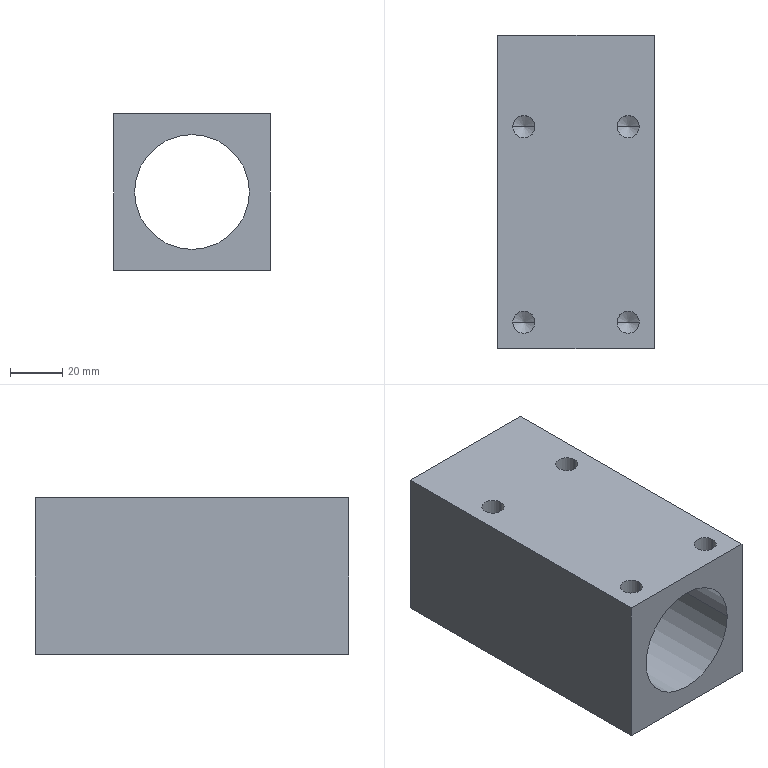Component | SolidWorks | -MovingBushing-3 | 1 solid | 40 faces | box 60 x 120 x 60 mm | volume 242794 mm3 | cylinder 18 | cone 16 | plane 6 | commonest cylinder face diameters 8.5 x16 44 x2
build123d program:
from build123d import *

# Parameters (mm, degrees)
SKETCH1_W                   = 60
SKETCH1_H                   = 60
SKETCH1_R                   = 22
BOSS_EXTRUDE1_DEPTH         = 60
M10_TAPPED_HOLE1_AT_2_COUNT = 2
M10_TAPPED_HOLE1_AT_2_PITCH = 40
M10_TAPPED_HOLE1_AT_3_COUNT = 2
M10_TAPPED_HOLE1_AT_3_PITCH = 75
M10_TAPPED_HOLE1_AT_4_COUNT = 2
M10_TAPPED_HOLE1_AT_4_PITCH = 85


with BuildPart() as part:
    # Sketch1 → Boss-Extrude1 (new, symmetric)
    with BuildSketch(Plane(origin=(0, 0, 0), x_dir=(0, 0, -1), z_dir=(1, 0, 0))):
        Rectangle(SKETCH1_W, SKETCH1_H)
        Circle(SKETCH1_R, mode=Mode.SUBTRACT)
    extrude(amount=BOSS_EXTRUDE1_DEPTH, both=True)

    # Sketch2 → M10 Tapped Hole1 (revolve, cut)
    with BuildSketch(Plane(origin=(-25, -30, 20), x_dir=(0, 0, -1), z_dir=(1, 0, 0))):
        Polygon((0, 0), (0, 16.554), (4.25, 14), (4.25, 0), align=None)
    m10_tapped_hole1 = revolve(axis=Axis((-25, -36.35, 20), (0, 1, 0)), mode=Mode.SUBTRACT)

    # M10 Tapped Hole1 at 2: M10 Tapped Hole1 ×2
    with Locations(*[(0, 0, -i * M10_TAPPED_HOLE1_AT_2_PITCH) for i in range(1, M10_TAPPED_HOLE1_AT_2_COUNT)]):
        add(m10_tapped_hole1, mode=Mode.SUBTRACT)

    # M10 Tapped Hole1 at 3: M10 Tapped Hole1 ×2
    with Locations(*[(i * M10_TAPPED_HOLE1_AT_3_PITCH, 0, 0) for i in range(1, M10_TAPPED_HOLE1_AT_3_COUNT)]):
        add(m10_tapped_hole1, mode=Mode.SUBTRACT)

    # M10 Tapped Hole1 at 4: M10 Tapped Hole1 ×2
    with Locations(*[Vector(0.8824, 0, -0.4706) * (i * M10_TAPPED_HOLE1_AT_4_PITCH) for i in range(1, M10_TAPPED_HOLE1_AT_4_COUNT)]):
        add(m10_tapped_hole1, mode=Mode.SUBTRACT)

    # Mirror1: M10 Tapped Hole1 across plane
    add(m10_tapped_hole1.mirror(Plane.ZX), mode=Mode.SUBTRACT)

    # Mirror1 copy 1 sketch → Mirror1 copy 1 (revolve, cut)
    with BuildSketch(Plane(origin=(-25, 30, -20), x_dir=(0, 0, -1), z_dir=(1, 0, 0))):
        Polygon((0, 0), (0, -16.554), (4.25, -14), (4.25, 0), align=None)
    revolve(axis=Axis((-25, 36.35, -20), (0, 1, 0)), mode=Mode.SUBTRACT)

    # Mirror1 copy 2 sketch → Mirror1 copy 2 (revolve, cut)
    with BuildSketch(Plane(origin=(50, 30, 20), x_dir=(0, 0, -1), z_dir=(1, 0, 0))):
        Polygon((0, 0), (0, -16.554), (4.25, -14), (4.25, 0), align=None)
    revolve(axis=Axis((50, 36.35, 20), (0, 1, 0)), mode=Mode.SUBTRACT)

    # Mirror1 copy 3 sketch → Mirror1 copy 3 (revolve, cut)
    with BuildSketch(Plane(origin=(50, 30, -20), x_dir=(0, 0, -1), z_dir=(1, 0, 0))):
        Polygon((0, 0), (0, -16.554), (4.25, -14), (4.25, 0), align=None)
    revolve(axis=Axis((50, 36.35, -20), (0, 1, 0)), mode=Mode.SUBTRACT)


solid = part.part

# Placed as in the assembly
solid = solid.moved(Location((-55, 1249.5, -40), (90, -90, 0)))
STEP:
#1=COLOUR_RGB('',0.7922,0.8196,0.9333);
#2=FILL_AREA_STYLE_COLOUR('',#1);
#3=FILL_AREA_STYLE('',(#2));
#4=SURFACE_STYLE_FILL_AREA(#3);
#5=SURFACE_SIDE_STYLE('',(#4));
#6=SURFACE_STYLE_USAGE(.BOTH.,#5);
#7=PRESENTATION_STYLE_ASSIGNMENT((#6));
#8=CARTESIAN_POINT('',(-1.545,50.177,-2.205));
#9=VERTEX_POINT('',#8);
#10=CARTESIAN_POINT('',(-1.211,50.177,-2.205));
#11=VERTEX_POINT('',#10);
#12=CARTESIAN_POINT('',(-1.378,50.177,-2.205));
#13=DIRECTION('',(-0.,-0.,-1.));
#14=DIRECTION('',(1.,0.,0.));
#15=AXIS2_PLACEMENT_3D('',#12,#13,#14);
#16=CIRCLE('',#15,0.1673);
#17=EDGE_CURVE('',#9,#11,#16,.T.);
#18=ORIENTED_EDGE('',*,*,#17,.F.);
#19=CARTESIAN_POINT('',(-1.545,50.177,-2.756));
#20=VERTEX_POINT('',#19);
#21=CARTESIAN_POINT('',(-1.545,50.177,-2.756));
#22=DIRECTION('',(-0.,-0.,-1.));
#23=VECTOR('',#22,39.37);
#24=LINE('',#21,#23);
#25=EDGE_CURVE('',#9,#20,#24,.T.);
#26=ORIENTED_EDGE('',*,*,#25,.T.);
#27=CARTESIAN_POINT('',(-1.211,50.177,-2.756));
#28=VERTEX_POINT('',#27);
#29=CARTESIAN_POINT('',(-1.378,50.177,-2.756));
#30=DIRECTION('',(-0.,-0.,-1.));
#31=DIRECTION('',(1.,0.,0.));
#32=AXIS2_PLACEMENT_3D('',#29,#30,#31);
#33=CIRCLE('',#32,0.1673);
#34=EDGE_CURVE('',#20,#28,#33,.T.);
#35=ORIENTED_EDGE('',*,*,#34,.T.);
#36=CARTESIAN_POINT('',(-1.211,50.177,-2.756));
#37=DIRECTION('',(-0.,-0.,-1.));
#38=VECTOR('',#37,39.37);
#39=LINE('',#36,#38);
#40=EDGE_CURVE('',#11,#28,#39,.T.);
#41=ORIENTED_EDGE('',*,*,#40,.F.);
#42=EDGE_LOOP('',(#18,#26,#35,#41));
#43=FACE_OUTER_BOUND('',#42,.T.);
#44=CARTESIAN_POINT('',(-1.378,50.177,-2.756));
#45=DIRECTION('',(-0.,-0.,-1.));
#46=DIRECTION('',(1.,0.,0.));
#47=AXIS2_PLACEMENT_3D('',#44,#45,#46);
#48=CYLINDRICAL_SURFACE('',#47,0.1673);
#49=ADVANCED_FACE('',(#43),#48,.F.);
#50=CARTESIAN_POINT('',(-1.378,50.177,-2.104));
#51=VERTEX_POINT('',#50);
#52=CARTESIAN_POINT('',(-1.211,50.177,-2.205));
#53=DIRECTION('',(0.8572,0.,-0.515));
#54=VECTOR('',#53,39.37);
#55=LINE('',#52,#54);
#56=EDGE_CURVE('',#51,#11,#55,.T.);
#57=ORIENTED_EDGE('',*,*,#56,.F.);
#58=CARTESIAN_POINT('',(-1.545,50.177,-2.205));
#59=DIRECTION('',(-0.8572,-0.,-0.515));
#60=VECTOR('',#59,39.37);
#61=LINE('',#58,#60);
#62=EDGE_CURVE('',#51,#9,#61,.T.);
#63=ORIENTED_EDGE('',*,*,#62,.T.);
#64=ORIENTED_EDGE('',*,*,#17,.T.);
#65=EDGE_LOOP('',(#57,#63,#64));
#66=FACE_OUTER_BOUND('',#65,.T.);
#67=CARTESIAN_POINT('',(-1.378,50.177,-2.205));
#68=DIRECTION('',(-0.,-0.,-1.));
#69=DIRECTION('',(1.,0.,0.));
#70=AXIS2_PLACEMENT_3D('',#67,#68,#69);
#71=CONICAL_SURFACE('',#70,0.1673,1.03);
#72=ADVANCED_FACE('',(#66),#71,.F.);
#73=CARTESIAN_POINT('',(-3.12,50.177,-2.205));
#74=VERTEX_POINT('',#73);
#75=CARTESIAN_POINT('',(-2.785,50.177,-2.205));
#76=VERTEX_POINT('',#75);
#77=CARTESIAN_POINT('',(-2.953,50.177,-2.205));
#78=DIRECTION('',(-0.,-0.,-1.));
#79=DIRECTION('',(1.,0.,0.));
#80=AXIS2_PLACEMENT_3D('',#77,#78,#79);
#81=CIRCLE('',#80,0.1673);
#82=EDGE_CURVE('',#74,#76,#81,.T.);
#83=ORIENTED_EDGE('',*,*,#82,.F.);
#84=CARTESIAN_POINT('',(-3.12,50.177,-2.756));
#85=VERTEX_POINT('',#84);
#86=CARTESIAN_POINT('',(-3.12,50.177,-2.756));
#87=DIRECTION('',(-0.,-0.,-1.));
#88=VECTOR('',#87,39.37);
#89=LINE('',#86,#88);
#90=EDGE_CURVE('',#74,#85,#89,.T.);
#91=ORIENTED_EDGE('',*,*,#90,.T.);
#92=CARTESIAN_POINT('',(-2.785,50.177,-2.756));
#93=VERTEX_POINT('',#92);
#94=CARTESIAN_POINT('',(-2.953,50.177,-2.756));
#95=DIRECTION('',(-0.,-0.,-1.));
#96=DIRECTION('',(1.,0.,0.));
#97=AXIS2_PLACEMENT_3D('',#94,#95,#96);
#98=CIRCLE('',#97,0.1673);
#99=EDGE_CURVE('',#85,#93,#98,.T.);
#100=ORIENTED_EDGE('',*,*,#99,.T.);
#101=CARTESIAN_POINT('',(-2.785,50.177,-2.756));
#102=DIRECTION('',(-0.,-0.,-1.));
#103=VECTOR('',#102,39.37);
#104=LINE('',#101,#103);
#105=EDGE_CURVE('',#76,#93,#104,.T.);
#106=ORIENTED_EDGE('',*,*,#105,.F.);
#107=EDGE_LOOP('',(#83,#91,#100,#106));
#108=FACE_OUTER_BOUND('',#107,.T.);
#109=CARTESIAN_POINT('',(-2.953,50.177,-2.756));
#110=DIRECTION('',(-0.,-0.,-1.));
#111=DIRECTION('',(1.,0.,0.));
#112=AXIS2_PLACEMENT_3D('',#109,#110,#111);
#113=CYLINDRICAL_SURFACE('',#112,0.1673);
#114=ADVANCED_FACE('',(#108),#113,.F.);
#115=CARTESIAN_POINT('',(-2.953,50.177,-2.104));
#116=VERTEX_POINT('',#115);
#117=CARTESIAN_POINT('',(-2.785,50.177,-2.205));
#118=DIRECTION('',(0.8572,0.,-0.515));
#119=VECTOR('',#118,39.37);
#120=LINE('',#117,#119);
#121=EDGE_CURVE('',#116,#76,#120,.T.);
#122=ORIENTED_EDGE('',*,*,#121,.F.);
#123=CARTESIAN_POINT('',(-3.12,50.177,-2.205));
#124=DIRECTION('',(-0.8572,-0.,-0.515));
#125=VECTOR('',#124,39.37);
#126=LINE('',#123,#125);
#127=EDGE_CURVE('',#116,#74,#126,.T.);
#128=ORIENTED_EDGE('',*,*,#127,.T.);
#129=ORIENTED_EDGE('',*,*,#82,.T.);
#130=EDGE_LOOP('',(#122,#128,#129));
#131=FACE_OUTER_BOUND('',#130,.T.);
#132=CARTESIAN_POINT('',(-2.953,50.177,-2.205));
#133=DIRECTION('',(-0.,-0.,-1.));
#134=DIRECTION('',(1.,0.,0.));
#135=AXIS2_PLACEMENT_3D('',#132,#133,#134);
#136=CONICAL_SURFACE('',#135,0.1673,1.03);
#137=ADVANCED_FACE('',(#131),#136,.F.);
#138=CARTESIAN_POINT('',(-1.545,47.224,-2.205));
#139=VERTEX_POINT('',#138);
#140=CARTESIAN_POINT('',(-1.211,47.224,-2.205));
#141=VERTEX_POINT('',#140);
#142=CARTESIAN_POINT('',(-1.378,47.224,-2.205));
#143=DIRECTION('',(-0.,-0.,-1.));
#144=DIRECTION('',(1.,0.,0.));
#145=AXIS2_PLACEMENT_3D('',#142,#143,#144);
#146=CIRCLE('',#145,0.1673);
#147=EDGE_CURVE('',#139,#141,#146,.T.);
#148=ORIENTED_EDGE('',*,*,#147,.F.);
#149=CARTESIAN_POINT('',(-1.545,47.224,-2.756));
#150=VERTEX_POINT('',#149);
#151=CARTESIAN_POINT('',(-1.545,47.224,-2.756));
#152=DIRECTION('',(-0.,-0.,-1.));
#153=VECTOR('',#152,39.37);
#154=LINE('',#151,#153);
#155=EDGE_CURVE('',#139,#150,#154,.T.);
#156=ORIENTED_EDGE('',*,*,#155,.T.);
#157=CARTESIAN_POINT('',(-1.211,47.224,-2.756));
#158=VERTEX_POINT('',#157);
#159=CARTESIAN_POINT('',(-1.378,47.224,-2.756));
#160=DIRECTION('',(-0.,-0.,-1.));
#161=DIRECTION('',(1.,0.,0.));
#162=AXIS2_PLACEMENT_3D('',#159,#160,#161);
#163=CIRCLE('',#162,0.1673);
#164=EDGE_CURVE('',#150,#158,#163,.T.);
#165=ORIENTED_EDGE('',*,*,#164,.T.);
#166=CARTESIAN_POINT('',(-1.211,47.224,-2.756));
#167=DIRECTION('',(-0.,-0.,-1.));
#168=VECTOR('',#167,39.37);
#169=LINE('',#166,#168);
#170=EDGE_CURVE('',#141,#158,#169,.T.);
#171=ORIENTED_EDGE('',*,*,#170,.F.);
#172=EDGE_LOOP('',(#148,#156,#165,#171));
#173=FACE_OUTER_BOUND('',#172,.T.);
#174=CARTESIAN_POINT('',(-1.378,47.224,-2.756));
#175=DIRECTION('',(-0.,-0.,-1.));
#176=DIRECTION('',(1.,0.,0.));
#177=AXIS2_PLACEMENT_3D('',#174,#175,#176);
#178=CYLINDRICAL_SURFACE('',#177,0.1673);
#179=ADVANCED_FACE('',(#173),#178,.F.);
#180=CARTESIAN_POINT('',(-1.378,47.224,-2.104));
#181=VERTEX_POINT('',#180);
#182=CARTESIAN_POINT('',(-1.211,47.224,-2.205));
#183=DIRECTION('',(0.8572,0.,-0.515));
#184=VECTOR('',#183,39.37);
#185=LINE('',#182,#184);
#186=EDGE_CURVE('',#181,#141,#185,.T.);
#187=ORIENTED_EDGE('',*,*,#186,.F.);
#188=CARTESIAN_POINT('',(-1.545,47.224,-2.205));
#189=DIRECTION('',(-0.8572,-0.,-0.515));
#190=VECTOR('',#189,39.37);
#191=LINE('',#188,#190);
#192=EDGE_CURVE('',#181,#139,#191,.T.);
#193=ORIENTED_EDGE('',*,*,#192,.T.);
#194=ORIENTED_EDGE('',*,*,#147,.T.);
#195=EDGE_LOOP('',(#187,#193,#194));
#196=FACE_OUTER_BOUND('',#195,.T.);
#197=CARTESIAN_POINT('',(-1.378,47.224,-2.205));
#198=DIRECTION('',(-0.,-0.,-1.));
#199=DIRECTION('',(1.,0.,0.));
#200=AXIS2_PLACEMENT_3D('',#197,#198,#199);
#201=CONICAL_SURFACE('',#200,0.1673,1.03);
#202=ADVANCED_FACE('',(#196),#201,.F.);
#203=CARTESIAN_POINT('',(-3.12,47.224,-2.205));
#204=VERTEX_POINT('',#203);
#205=CARTESIAN_POINT('',(-2.785,47.224,-2.205));
#206=VERTEX_POINT('',#205);
#207=CARTESIAN_POINT('',(-2.953,47.224,-2.205));
#208=DIRECTION('',(-0.,-0.,-1.));
#209=DIRECTION('',(1.,0.,0.));
#210=AXIS2_PLACEMENT_3D('',#207,#208,#209);
#211=CIRCLE('',#210,0.1673);
#212=EDGE_CURVE('',#204,#206,#211,.T.);
#213=ORIENTED_EDGE('',*,*,#212,.F.);
#214=CARTESIAN_POINT('',(-3.12,47.224,-2.756));
#215=VERTEX_POINT('',#214);
#216=CARTESIAN_POINT('',(-3.12,47.224,-2.756));
#217=DIRECTION('',(-0.,-0.,-1.));
#218=VECTOR('',#217,39.37);
#219=LINE('',#216,#218);
#220=EDGE_CURVE('',#204,#215,#219,.T.);
#221=ORIENTED_EDGE('',*,*,#220,.T.);
#222=CARTESIAN_POINT('',(-2.785,47.224,-2.756));
#223=VERTEX_POINT('',#222);
#224=CARTESIAN_POINT('',(-2.953,47.224,-2.756));
#225=DIRECTION('',(-0.,-0.,-1.));
#226=DIRECTION('',(1.,0.,0.));
#227=AXIS2_PLACEMENT_3D('',#224,#225,#226);
#228=CIRCLE('',#227,0.1673);
#229=EDGE_CURVE('',#215,#223,#228,.T.);
#230=ORIENTED_EDGE('',*,*,#229,.T.);
#231=CARTESIAN_POINT('',(-2.785,47.224,-2.756));
#232=DIRECTION('',(-0.,-0.,-1.));
#233=VECTOR('',#232,39.37);
#234=LINE('',#231,#233);
#235=EDGE_CURVE('',#206,#223,#234,.T.);
#236=ORIENTED_EDGE('',*,*,#235,.F.);
#237=EDGE_LOOP('',(#213,#221,#230,#236));
#238=FACE_OUTER_BOUND('',#237,.T.);
#239=CARTESIAN_POINT('',(-2.953,47.224,-2.756));
#240=DIRECTION('',(-0.,-0.,-1.));
#241=DIRECTION('',(1.,0.,0.));
#242=AXIS2_PLACEMENT_3D('',#239,#240,#241);
#243=CYLINDRICAL_SURFACE('',#242,0.1673);
#244=ADVANCED_FACE('',(#238),#243,.F.);
#245=CARTESIAN_POINT('',(-2.953,47.224,-2.104));
#246=VERTEX_POINT('',#245);
#247=CARTESIAN_POINT('',(-2.785,47.224,-2.205));
#248=DIRECTION('',(0.8572,0.,-0.515));
#249=VECTOR('',#248,39.37);
#250=LINE('',#247,#249);
#251=EDGE_CURVE('',#246,#206,#250,.T.);
#252=ORIENTED_EDGE('',*,*,#251,.F.);
#253=CARTESIAN_POINT('',(-3.12,47.224,-2.205));
#254=DIRECTION('',(-0.8572,-0.,-0.515));
#255=VECTOR('',#254,39.37);
#256=LINE('',#253,#255);
#257=EDGE_CURVE('',#246,#204,#256,.T.);
#258=ORIENTED_EDGE('',*,*,#257,.T.);
#259=ORIENTED_EDGE('',*,*,#212,.T.);
#260=EDGE_LOOP('',(#252,#258,#259));
#261=FACE_OUTER_BOUND('',#260,.T.);
#262=CARTESIAN_POINT('',(-2.953,47.224,-2.205));
#263=DIRECTION('',(-0.,-0.,-1.));
#264=DIRECTION('',(1.,0.,0.));
#265=AXIS2_PLACEMENT_3D('',#262,#263,#264);
#266=CONICAL_SURFACE('',#265,0.1673,1.03);
#267=ADVANCED_FACE('',(#261),#266,.F.);
#268=CARTESIAN_POINT('',(-1.211,50.177,-0.9449));
#269=VERTEX_POINT('',#268);
#270=CARTESIAN_POINT('',(-1.545,50.177,-0.9449));
#271=VERTEX_POINT('',#270);
#272=CARTESIAN_POINT('',(-1.378,50.177,-0.9449));
#273=DIRECTION('',(0.,0.,1.));
#274=DIRECTION('',(-1.,0.,0.));
#275=AXIS2_PLACEMENT_3D('',#272,#273,#274);
#276=CIRCLE('',#275,0.1673);
#277=EDGE_CURVE('',#269,#271,#276,.T.);
#278=ORIENTED_EDGE('',*,*,#277,.F.);
#279=CARTESIAN_POINT('',(-1.211,50.177,-0.3937));
#280=VERTEX_POINT('',#279);
#281=CARTESIAN_POINT('',(-1.211,50.177,-0.3937));
#282=DIRECTION('',(0.,0.,1.));
#283=VECTOR('',#282,39.37);
#284=LINE('',#281,#283);
#285=EDGE_CURVE('',#269,#280,#284,.T.);
#286=ORIENTED_EDGE('',*,*,#285,.T.);
#287=CARTESIAN_POINT('',(-1.545,50.177,-0.3937));
#288=VERTEX_POINT('',#287);
#289=CARTESIAN_POINT('',(-1.378,50.177,-0.3937));
#290=DIRECTION('',(0.,0.,1.));
#291=DIRECTION('',(-1.,0.,0.));
#292=AXIS2_PLACEMENT_3D('',#289,#290,#291);
#293=CIRCLE('',#292,0.1673);
#294=EDGE_CURVE('',#280,#288,#293,.T.);
#295=ORIENTED_EDGE('',*,*,#294,.T.);
#296=CARTESIAN_POINT('',(-1.545,50.177,-0.3937));
#297=DIRECTION('',(0.,0.,1.));
#298=VECTOR('',#297,39.37);
#299=LINE('',#296,#298);
#300=EDGE_CURVE('',#271,#288,#299,.T.);
#301=ORIENTED_EDGE('',*,*,#300,.F.);
#302=EDGE_LOOP('',(#278,#286,#295,#301));
#303=FACE_OUTER_BOUND('',#302,.T.);
#304=CARTESIAN_POINT('',(-1.378,50.177,-0.3937));
#305=DIRECTION('',(0.,0.,1.));
#306=DIRECTION('',(-1.,0.,0.));
#307=AXIS2_PLACEMENT_3D('',#304,#305,#306);
#308=CYLINDRICAL_SURFACE('',#307,0.1673);
#309=ADVANCED_FACE('',(#303),#308,.F.);
#310=CARTESIAN_POINT('',(-1.378,50.177,-1.045));
#311=VERTEX_POINT('',#310);
#312=CARTESIAN_POINT('',(-1.545,50.177,-0.9449));
#313=DIRECTION('',(-0.8572,-0.,0.515));
#314=VECTOR('',#313,39.37);
#315=LINE('',#312,#314);
#316=EDGE_CURVE('',#311,#271,#315,.T.);
#317=ORIENTED_EDGE('',*,*,#316,.F.);
#318=CARTESIAN_POINT('',(-1.211,50.177,-0.9449));
#319=DIRECTION('',(0.8572,0.,0.515));
#320=VECTOR('',#319,39.37);
#321=LINE('',#318,#320);
#322=EDGE_CURVE('',#311,#269,#321,.T.);
#323=ORIENTED_EDGE('',*,*,#322,.T.);
#324=ORIENTED_EDGE('',*,*,#277,.T.);
#325=EDGE_LOOP('',(#317,#323,#324));
#326=FACE_OUTER_BOUND('',#325,.T.);
#327=CARTESIAN_POINT('',(-1.378,50.177,-0.9449));
#328=DIRECTION('',(0.,0.,1.));
#329=DIRECTION('',(-1.,0.,0.));
#330=AXIS2_PLACEMENT_3D('',#327,#328,#329);
#331=CONICAL_SURFACE('',#330,0.1673,1.03);
#332=ADVANCED_FACE('',(#326),#331,.F.);
#333=CARTESIAN_POINT('',(-2.785,50.177,-0.9449));
#334=VERTEX_POINT('',#333);
#335=CARTESIAN_POINT('',(-3.12,50.177,-0.9449));
#336=VERTEX_POINT('',#335);
#337=CARTESIAN_POINT('',(-2.953,50.177,-0.9449));
#338=DIRECTION('',(0.,0.,1.));
#339=DIRECTION('',(-1.,0.,0.));
#340=AXIS2_PLACEMENT_3D('',#337,#338,#339);
#341=CIRCLE('',#340,0.1673);
#342=EDGE_CURVE('',#334,#336,#341,.T.);
#343=ORIENTED_EDGE('',*,*,#342,.F.);
#344=CARTESIAN_POINT('',(-2.785,50.177,-0.3937));
#345=VERTEX_POINT('',#344);
#346=CARTESIAN_POINT('',(-2.785,50.177,-0.3937));
#347=DIRECTION('',(0.,0.,1.));
#348=VECTOR('',#347,39.37);
#349=LINE('',#346,#348);
#350=EDGE_CURVE('',#334,#345,#349,.T.);
#351=ORIENTED_EDGE('',*,*,#350,.T.);
#352=CARTESIAN_POINT('',(-3.12,50.177,-0.3937));
#353=VERTEX_POINT('',#352);
#354=CARTESIAN_POINT('',(-2.953,50.177,-0.3937));
#355=DIRECTION('',(0.,0.,1.));
#356=DIRECTION('',(-1.,0.,0.));
#357=AXIS2_PLACEMENT_3D('',#354,#355,#356);
#358=CIRCLE('',#357,0.1673);
#359=EDGE_CURVE('',#345,#353,#358,.T.);
#360=ORIENTED_EDGE('',*,*,#359,.T.);
#361=CARTESIAN_POINT('',(-3.12,50.177,-0.3937));
#362=DIRECTION('',(0.,0.,1.));
#363=VECTOR('',#362,39.37);
#364=LINE('',#361,#363);
#365=EDGE_CURVE('',#336,#353,#364,.T.);
#366=ORIENTED_EDGE('',*,*,#365,.F.);
#367=EDGE_LOOP('',(#343,#351,#360,#366));
#368=FACE_OUTER_BOUND('',#367,.T.);
#369=CARTESIAN_POINT('',(-2.953,50.177,-0.3937));
#370=DIRECTION('',(0.,0.,1.));
#371=DIRECTION('',(-1.,0.,0.));
#372=AXIS2_PLACEMENT_3D('',#369,#370,#371);
#373=CYLINDRICAL_SURFACE('',#372,0.1673);
#374=ADVANCED_FACE('',(#368),#373,.F.);
#375=CARTESIAN_POINT('',(-2.953,50.177,-1.045));
#376=VERTEX_POINT('',#375);
#377=CARTESIAN_POINT('',(-3.12,50.177,-0.9449));
#378=DIRECTION('',(-0.8572,-0.,0.515));
#379=VECTOR('',#378,39.37);
#380=LINE('',#377,#379);
#381=EDGE_CURVE('',#376,#336,#380,.T.);
#382=ORIENTED_EDGE('',*,*,#381,.F.);
#383=CARTESIAN_POINT('',(-2.785,50.177,-0.9449));
#384=DIRECTION('',(0.8572,0.,0.515));
#385=VECTOR('',#384,39.37);
#386=LINE('',#383,#385);
#387=EDGE_CURVE('',#376,#334,#386,.T.);
#388=ORIENTED_EDGE('',*,*,#387,.T.);
#389=ORIENTED_EDGE('',*,*,#342,.T.);
#390=EDGE_LOOP('',(#382,#388,#389));
#391=FACE_OUTER_BOUND('',#390,.T.);
#392=CARTESIAN_POINT('',(-2.953,50.177,-0.9449));
#393=DIRECTION('',(0.,0.,1.));
#394=DIRECTION('',(-1.,0.,0.));
#395=AXIS2_PLACEMENT_3D('',#392,#393,#394);
#396=CONICAL_SURFACE('',#395,0.1673,1.03);
#397=ADVANCED_FACE('',(#391),#396,.F.);
#398=CARTESIAN_POINT('',(-1.211,47.224,-0.9449));
#399=VERTEX_POINT('',#398);
#400=CARTESIAN_POINT('',(-1.545,47.224,-0.9449));
#401=VERTEX_POINT('',#400);
#402=CARTESIAN_POINT('',(-1.378,47.224,-0.9449));
#403=DIRECTION('',(0.,0.,1.));
#404=DIRECTION('',(-1.,0.,0.));
#405=AXIS2_PLACEMENT_3D('',#402,#403,#404);
#406=CIRCLE('',#405,0.1673);
#407=EDGE_CURVE('',#399,#401,#406,.T.);
#408=ORIENTED_EDGE('',*,*,#407,.F.);
#409=CARTESIAN_POINT('',(-1.211,47.224,-0.3937));
#410=VERTEX_POINT('',#409);
#411=CARTESIAN_POINT('',(-1.211,47.224,-0.3937));
#412=DIRECTION('',(0.,0.,1.));
#413=VECTOR('',#412,39.37);
#414=LINE('',#411,#413);
#415=EDGE_CURVE('',#399,#410,#414,.T.);
#416=ORIENTED_EDGE('',*,*,#415,.T.);
#417=CARTESIAN_POINT('',(-1.545,47.224,-0.3937));
#418=VERTEX_POINT('',#417);
#419=CARTESIAN_POINT('',(-1.378,47.224,-0.3937));
#420=DIRECTION('',(0.,0.,1.));
#421=DIRECTION('',(-1.,0.,0.));
#422=AXIS2_PLACEMENT_3D('',#419,#420,#421);
#423=CIRCLE('',#422,0.1673);
#424=EDGE_CURVE('',#410,#418,#423,.T.);
#425=ORIENTED_EDGE('',*,*,#424,.T.);
#426=CARTESIAN_POINT('',(-1.545,47.224,-0.3937));
#427=DIRECTION('',(0.,0.,1.));
#428=VECTOR('',#427,39.37);
#429=LINE('',#426,#428);
#430=EDGE_CURVE('',#401,#418,#429,.T.);
#431=ORIENTED_EDGE('',*,*,#430,.F.);
#432=EDGE_LOOP('',(#408,#416,#425,#431));
#433=FACE_OUTER_BOUND('',#432,.T.);
#434=CARTESIAN_POINT('',(-1.378,47.224,-0.3937));
#435=DIRECTION('',(0.,0.,1.));
#436=DIRECTION('',(-1.,0.,0.));
#437=AXIS2_PLACEMENT_3D('',#434,#435,#436);
#438=CYLINDRICAL_SURFACE('',#437,0.1673);
#439=ADVANCED_FACE('',(#433),#438,.F.);
#440=CARTESIAN_POINT('',(-1.378,47.224,-1.045));
#441=VERTEX_POINT('',#440);
#442=CARTESIAN_POINT('',(-1.545,47.224,-0.9449));
#443=DIRECTION('',(-0.8572,-0.,0.515));
#444=VECTOR('',#443,39.37);
#445=LINE('',#442,#444);
#446=EDGE_CURVE('',#441,#401,#445,.T.);
#447=ORIENTED_EDGE('',*,*,#446,.F.);
#448=CARTESIAN_POINT('',(-1.211,47.224,-0.9449));
#449=DIRECTION('',(0.8572,0.,0.515));
#450=VECTOR('',#449,39.37);
#451=LINE('',#448,#450);
#452=EDGE_CURVE('',#441,#399,#451,.T.);
#453=ORIENTED_EDGE('',*,*,#452,.T.);
#454=ORIENTED_EDGE('',*,*,#407,.T.);
#455=EDGE_LOOP('',(#447,#453,#454));
#456=FACE_OUTER_BOUND('',#455,.T.);
#457=CARTESIAN_POINT('',(-1.378,47.224,-0.9449));
#458=DIRECTION('',(0.,0.,1.));
#459=DIRECTION('',(-1.,0.,0.));
#460=AXIS2_PLACEMENT_3D('',#457,#458,#459);
#461=CONICAL_SURFACE('',#460,0.1673,1.03);
#462=ADVANCED_FACE('',(#456),#461,.F.);
#463=CARTESIAN_POINT('',(-2.785,47.224,-0.9449));
#464=VERTEX_POINT('',#463);
#465=CARTESIAN_POINT('',(-3.12,47.224,-0.9449));
#466=VERTEX_POINT('',#465);
#467=CARTESIAN_POINT('',(-2.953,47.224,-0.9449));
#468=DIRECTION('',(0.,0.,1.));
#469=DIRECTION('',(-1.,0.,0.));
#470=AXIS2_PLACEMENT_3D('',#467,#468,#469);
#471=CIRCLE('',#470,0.1673);
#472=EDGE_CURVE('',#464,#466,#471,.T.);
#473=ORIENTED_EDGE('',*,*,#472,.F.);
#474=CARTESIAN_POINT('',(-2.785,47.224,-0.3937));
#475=VERTEX_POINT('',#474);
#476=CARTESIAN_POINT('',(-2.785,47.224,-0.3937));
#477=DIRECTION('',(0.,0.,1.));
#478=VECTOR('',#477,39.37);
#479=LINE('',#476,#478);
#480=EDGE_CURVE('',#464,#475,#479,.T.);
#481=ORIENTED_EDGE('',*,*,#480,.T.);
#482=CARTESIAN_POINT('',(-3.12,47.224,-0.3937));
#483=VERTEX_POINT('',#482);
#484=CARTESIAN_POINT('',(-2.953,47.224,-0.3937));
#485=DIRECTION('',(0.,0.,1.));
#486=DIRECTION('',(-1.,0.,0.));
#487=AXIS2_PLACEMENT_3D('',#484,#485,#486);
#488=CIRCLE('',#487,0.1673);
#489=EDGE_CURVE('',#475,#483,#488,.T.);
#490=ORIENTED_EDGE('',*,*,#489,.T.);
#491=CARTESIAN_POINT('',(-3.12,47.224,-0.3937));
#492=DIRECTION('',(0.,0.,1.));
#493=VECTOR('',#492,39.37);
#494=LINE('',#491,#493);
#495=EDGE_CURVE('',#466,#483,#494,.T.);
#496=ORIENTED_EDGE('',*,*,#495,.F.);
#497=EDGE_LOOP('',(#473,#481,#490,#496));
#498=FACE_OUTER_BOUND('',#497,.T.);
#499=CARTESIAN_POINT('',(-2.953,47.224,-0.3937));
#500=DIRECTION('',(0.,0.,1.));
#501=DIRECTION('',(-1.,0.,0.));
#502=AXIS2_PLACEMENT_3D('',#499,#500,#501);
#503=CYLINDRICAL_SURFACE('',#502,0.1673);
#504=ADVANCED_FACE('',(#498),#503,.F.);
#505=CARTESIAN_POINT('',(-2.953,47.224,-1.045));
#506=VERTEX_POINT('',#505);
#507=CARTESIAN_POINT('',(-3.12,47.224,-0.9449));
#508=DIRECTION('',(-0.8572,-0.,0.515));
#509=VECTOR('',#508,39.37);
#510=LINE('',#507,#509);
#511=EDGE_CURVE('',#506,#466,#510,.T.);
#512=ORIENTED_EDGE('',*,*,#511,.F.);
#513=CARTESIAN_POINT('',(-2.785,47.224,-0.9449));
#514=DIRECTION('',(0.8572,0.,0.515));
#515=VECTOR('',#514,39.37);
#516=LINE('',#513,#515);
#517=EDGE_CURVE('',#506,#464,#516,.T.);
#518=ORIENTED_EDGE('',*,*,#517,.T.);
#519=ORIENTED_EDGE('',*,*,#472,.T.);
#520=EDGE_LOOP('',(#512,#518,#519));
#521=FACE_OUTER_BOUND('',#520,.T.);
#522=CARTESIAN_POINT('',(-2.953,47.224,-0.9449));
#523=DIRECTION('',(0.,0.,1.));
#524=DIRECTION('',(-1.,0.,0.));
#525=AXIS2_PLACEMENT_3D('',#522,#523,#524);
#526=CONICAL_SURFACE('',#525,0.1673,1.03);
#527=ADVANCED_FACE('',(#521),#526,.F.);
#528=CARTESIAN_POINT('',(-1.299,46.831,-1.575));
#529=VERTEX_POINT('',#528);
#530=CARTESIAN_POINT('',(-3.031,46.831,-1.575));
#531=VERTEX_POINT('',#530);
#532=CARTESIAN_POINT('',(-2.165,46.831,-1.575));
#533=DIRECTION('',(0.,-1.,0.));
#534=DIRECTION('',(-1.,-0.,0.));
#535=AXIS2_PLACEMENT_3D('',#532,#533,#534);
#536=CIRCLE('',#535,0.8661);
#537=EDGE_CURVE('',#529,#531,#536,.T.);
#538=ORIENTED_EDGE('',*,*,#537,.T.);
#539=CARTESIAN_POINT('',(-3.031,51.555,-1.575));
#540=VERTEX_POINT('',#539);
#541=CARTESIAN_POINT('',(-3.031,46.831,-1.575));
#542=DIRECTION('',(-0.,1.,-0.));
#543=VECTOR('',#542,39.37);
#544=LINE('',#541,#543);
#545=EDGE_CURVE('',#531,#540,#544,.T.);
#546=ORIENTED_EDGE('',*,*,#545,.T.);
#547=CARTESIAN_POINT('',(-1.299,51.555,-1.575));
#548=VERTEX_POINT('',#547);
#549=CARTESIAN_POINT('',(-2.165,51.555,-1.575));
#550=DIRECTION('',(0.,-1.,0.));
#551=DIRECTION('',(-1.,-0.,0.));
#552=AXIS2_PLACEMENT_3D('',#549,#550,#551);
#553=CIRCLE('',#552,0.8661);
#554=EDGE_CURVE('',#548,#540,#553,.T.);
#555=ORIENTED_EDGE('',*,*,#554,.F.);
#556=CARTESIAN_POINT('',(-1.299,46.831,-1.575));
#557=DIRECTION('',(-0.,1.,-0.));
#558=VECTOR('',#557,39.37);
#559=LINE('',#556,#558);
#560=EDGE_CURVE('',#529,#548,#559,.T.);
#561=ORIENTED_EDGE('',*,*,#560,.F.);
#562=EDGE_LOOP('',(#538,#546,#555,#561));
#563=FACE_OUTER_BOUND('',#562,.T.);
#564=CARTESIAN_POINT('',(-2.165,46.831,-1.575));
#565=DIRECTION('',(-0.,1.,-0.));
#566=DIRECTION('',(1.,0.,-0.));
#567=AXIS2_PLACEMENT_3D('',#564,#565,#566);
#568=CYLINDRICAL_SURFACE('',#567,0.8661);
#569=ADVANCED_FACE('',(#563),#568,.F.);
#570=CARTESIAN_POINT('',(-3.346,46.831,-0.3937));
#571=VERTEX_POINT('',#570);
#572=CARTESIAN_POINT('',(-3.346,46.831,-2.756));
#573=VERTEX_POINT('',#572);
#574=CARTESIAN_POINT('',(-3.346,46.831,-2.756));
#575=DIRECTION('',(-0.,-0.,-1.));
#576=VECTOR('',#575,39.37);
#577=LINE('',#574,#576);
#578=EDGE_CURVE('',#571,#573,#577,.T.);
#579=ORIENTED_EDGE('',*,*,#578,.T.);
#580=CARTESIAN_POINT('',(-0.9843,46.831,-2.756));
#581=VERTEX_POINT('',#580);
#582=CARTESIAN_POINT('',(-0.9843,46.831,-2.756));
#583=DIRECTION('',(1.,0.,-0.));
#584=VECTOR('',#583,39.37);
#585=LINE('',#582,#584);
#586=EDGE_CURVE('',#573,#581,#585,.T.);
#587=ORIENTED_EDGE('',*,*,#586,.T.);
#588=CARTESIAN_POINT('',(-0.9843,46.831,-0.3937));
#589=VERTEX_POINT('',#588);
#590=CARTESIAN_POINT('',(-0.9843,46.831,-2.756));
#591=DIRECTION('',(0.,0.,1.));
#592=VECTOR('',#591,39.37);
#593=LINE('',#590,#592);
#594=EDGE_CURVE('',#581,#589,#593,.T.);
#595=ORIENTED_EDGE('',*,*,#594,.T.);
#596=CARTESIAN_POINT('',(-0.9843,46.831,-0.3937));
#597=DIRECTION('',(-1.,-0.,0.));
#598=VECTOR('',#597,39.37);
#599=LINE('',#596,#598);
#600=EDGE_CURVE('',#589,#571,#599,.T.);
#601=ORIENTED_EDGE('',*,*,#600,.T.);
#602=EDGE_LOOP('',(#579,#587,#595,#601));
#603=FACE_OUTER_BOUND('',#602,.T.);
#604=ORIENTED_EDGE('',*,*,#537,.F.);
#605=CARTESIAN_POINT('',(-2.165,46.831,-1.575));
#606=DIRECTION('',(0.,-1.,0.));
#607=DIRECTION('',(-1.,-0.,0.));
#608=AXIS2_PLACEMENT_3D('',#605,#606,#607);
#609=CIRCLE('',#608,0.8661);
#610=EDGE_CURVE('',#531,#529,#609,.T.);
#611=ORIENTED_EDGE('',*,*,#610,.F.);
#612=EDGE_LOOP('',(#604,#611));
#613=FACE_BOUND('',#612,.T.);
#614=CARTESIAN_POINT('',(-2.165,46.831,-1.575));
#615=DIRECTION('',(0.,-1.,0.));
#616=DIRECTION('',(-1.,-0.,0.));
#617=AXIS2_PLACEMENT_3D('',#614,#615,#616);
#618=PLANE('',#617);
#619=ADVANCED_FACE('',(#603,#613),#618,.T.);
#620=CARTESIAN_POINT('',(-3.346,51.555,-0.3937));
#621=VERTEX_POINT('',#620);
#622=CARTESIAN_POINT('',(-3.346,51.555,-2.756));
#623=VERTEX_POINT('',#622);
#624=CARTESIAN_POINT('',(-3.346,51.555,-2.756));
#625=DIRECTION('',(-0.,-0.,-1.));
#626=VECTOR('',#625,39.37);
#627=LINE('',#624,#626);
#628=EDGE_CURVE('',#621,#623,#627,.T.);
#629=ORIENTED_EDGE('',*,*,#628,.F.);
#630=CARTESIAN_POINT('',(-0.9843,51.555,-0.3937));
#631=VERTEX_POINT('',#630);
#632=CARTESIAN_POINT('',(-0.9843,51.555,-0.3937));
#633=DIRECTION('',(-1.,-0.,0.));
#634=VECTOR('',#633,39.37);
#635=LINE('',#632,#634);
#636=EDGE_CURVE('',#631,#621,#635,.T.);
#637=ORIENTED_EDGE('',*,*,#636,.F.);
#638=CARTESIAN_POINT('',(-0.9843,51.555,-2.756));
#639=VERTEX_POINT('',#638);
#640=CARTESIAN_POINT('',(-0.9843,51.555,-2.756));
#641=DIRECTION('',(0.,0.,1.));
#642=VECTOR('',#641,39.37);
#643=LINE('',#640,#642);
#644=EDGE_CURVE('',#639,#631,#643,.T.);
#645=ORIENTED_EDGE('',*,*,#644,.F.);
#646=CARTESIAN_POINT('',(-0.9843,51.555,-2.756));
#647=DIRECTION('',(1.,0.,-0.));
#648=VECTOR('',#647,39.37);
#649=LINE('',#646,#648);
#650=EDGE_CURVE('',#623,#639,#649,.T.);
#651=ORIENTED_EDGE('',*,*,#650,.F.);
#652=EDGE_LOOP('',(#629,#637,#645,#651));
#653=FACE_OUTER_BOUND('',#652,.T.);
#654=ORIENTED_EDGE('',*,*,#554,.T.);
#655=CARTESIAN_POINT('',(-2.165,51.555,-1.575));
#656=DIRECTION('',(0.,-1.,0.));
#657=DIRECTION('',(-1.,-0.,0.));
#658=AXIS2_PLACEMENT_3D('',#655,#656,#657);
#659=CIRCLE('',#658,0.8661);
#660=EDGE_CURVE('',#540,#548,#659,.T.);
#661=ORIENTED_EDGE('',*,*,#660,.T.);
#662=EDGE_LOOP('',(#654,#661));
#663=FACE_BOUND('',#662,.T.);
#664=CARTESIAN_POINT('',(-2.165,51.555,-1.575));
#665=DIRECTION('',(0.,-1.,0.));
#666=DIRECTION('',(-1.,-0.,0.));
#667=AXIS2_PLACEMENT_3D('',#664,#665,#666);
#668=PLANE('',#667);
#669=ADVANCED_FACE('',(#653,#663),#668,.F.);
#670=ORIENTED_EDGE('',*,*,#628,.T.);
#671=CARTESIAN_POINT('',(-3.346,46.831,-2.756));
#672=DIRECTION('',(-0.,1.,-0.));
#673=VECTOR('',#672,39.37);
#674=LINE('',#671,#673);
#675=EDGE_CURVE('',#573,#623,#674,.T.);
#676=ORIENTED_EDGE('',*,*,#675,.F.);
#677=ORIENTED_EDGE('',*,*,#578,.F.);
#678=CARTESIAN_POINT('',(-3.346,46.831,-0.3937));
#679=DIRECTION('',(-0.,1.,-0.));
#680=VECTOR('',#679,39.37);
#681=LINE('',#678,#680);
#682=EDGE_CURVE('',#571,#621,#681,.T.);
#683=ORIENTED_EDGE('',*,*,#682,.T.);
#684=EDGE_LOOP('',(#670,#676,#677,#683));
#685=FACE_OUTER_BOUND('',#684,.T.);
#686=CARTESIAN_POINT('',(-3.346,46.831,-2.756));
#687=DIRECTION('',(1.,0.,-0.));
#688=DIRECTION('',(0.,0.,1.));
#689=AXIS2_PLACEMENT_3D('',#686,#687,#688);
#690=PLANE('',#689);
#691=ADVANCED_FACE('',(#685),#690,.F.);
#692=CARTESIAN_POINT('',(-1.378,50.177,-2.756));
#693=DIRECTION('',(-0.,-0.,-1.));
#694=DIRECTION('',(1.,0.,0.));
#695=AXIS2_PLACEMENT_3D('',#692,#693,#694);
#696=CIRCLE('',#695,0.1673);
#697=EDGE_CURVE('',#28,#20,#696,.T.);
#698=ORIENTED_EDGE('',*,*,#697,.F.);
#699=ORIENTED_EDGE('',*,*,#34,.F.);
#700=EDGE_LOOP('',(#698,#699));
#701=FACE_BOUND('',#700,.T.);
#702=CARTESIAN_POINT('',(-2.953,50.177,-2.756));
#703=DIRECTION('',(-0.,-0.,-1.));
#704=DIRECTION('',(1.,0.,0.));
#705=AXIS2_PLACEMENT_3D('',#702,#703,#704);
#706=CIRCLE('',#705,0.1673);
#707=EDGE_CURVE('',#93,#85,#706,.T.);
#708=ORIENTED_EDGE('',*,*,#707,.F.);
#709=ORIENTED_EDGE('',*,*,#99,.F.);
#710=EDGE_LOOP('',(#708,#709));
#711=FACE_BOUND('',#710,.T.);
#712=CARTESIAN_POINT('',(-1.378,47.224,-2.756));
#713=DIRECTION('',(-0.,-0.,-1.));
#714=DIRECTION('',(1.,0.,0.));
#715=AXIS2_PLACEMENT_3D('',#712,#713,#714);
#716=CIRCLE('',#715,0.1673);
#717=EDGE_CURVE('',#158,#150,#716,.T.);
#718=ORIENTED_EDGE('',*,*,#717,.F.);
#719=ORIENTED_EDGE('',*,*,#164,.F.);
#720=EDGE_LOOP('',(#718,#719));
#721=FACE_BOUND('',#720,.T.);
#722=CARTESIAN_POINT('',(-2.953,47.224,-2.756));
#723=DIRECTION('',(-0.,-0.,-1.));
#724=DIRECTION('',(1.,0.,0.));
#725=AXIS2_PLACEMENT_3D('',#722,#723,#724);
#726=CIRCLE('',#725,0.1673);
#727=EDGE_CURVE('',#223,#215,#726,.T.);
#728=ORIENTED_EDGE('',*,*,#727,.F.);
#729=ORIENTED_EDGE('',*,*,#229,.F.);
#730=EDGE_LOOP('',(#728,#729));
#731=FACE_BOUND('',#730,.T.);
#732=ORIENTED_EDGE('',*,*,#650,.T.);
#733=CARTESIAN_POINT('',(-0.9843,46.831,-2.756));
#734=DIRECTION('',(-0.,1.,-0.));
#735=VECTOR('',#734,39.37);
#736=LINE('',#733,#735);
#737=EDGE_CURVE('',#581,#639,#736,.T.);
#738=ORIENTED_EDGE('',*,*,#737,.F.);
#739=ORIENTED_EDGE('',*,*,#586,.F.);
#740=ORIENTED_EDGE('',*,*,#675,.T.);
#741=EDGE_LOOP('',(#732,#738,#739,#740));
#742=FACE_OUTER_BOUND('',#741,.T.);
#743=CARTESIAN_POINT('',(-0.9843,46.831,-2.756));
#744=DIRECTION('',(0.,0.,1.));
#745=DIRECTION('',(-1.,-0.,0.));
#746=AXIS2_PLACEMENT_3D('',#743,#744,#745);
#747=PLANE('',#746);
#748=ADVANCED_FACE('',(#701,#711,#721,#731,#742),#747,.F.);
#749=ORIENTED_EDGE('',*,*,#644,.T.);
#750=CARTESIAN_POINT('',(-0.9843,46.831,-0.3937));
#751=DIRECTION('',(-0.,1.,-0.));
#752=VECTOR('',#751,39.37);
#753=LINE('',#750,#752);
#754=EDGE_CURVE('',#589,#631,#753,.T.);
#755=ORIENTED_EDGE('',*,*,#754,.F.);
#756=ORIENTED_EDGE('',*,*,#594,.F.);
#757=ORIENTED_EDGE('',*,*,#737,.T.);
#758=EDGE_LOOP('',(#749,#755,#756,#757));
#759=FACE_OUTER_BOUND('',#758,.T.);
#760=CARTESIAN_POINT('',(-0.9843,46.831,-2.756));
#761=DIRECTION('',(-1.,-0.,0.));
#762=DIRECTION('',(-0.,-0.,-1.));
#763=AXIS2_PLACEMENT_3D('',#760,#761,#762);
#764=PLANE('',#763);
#765=ADVANCED_FACE('',(#759),#764,.F.);
#766=CARTESIAN_POINT('',(-1.378,50.177,-0.3937));
#767=DIRECTION('',(0.,0.,1.));
#768=DIRECTION('',(-1.,0.,0.));
#769=AXIS2_PLACEMENT_3D('',#766,#767,#768);
#770=CIRCLE('',#769,0.1673);
#771=EDGE_CURVE('',#288,#280,#770,.T.);
#772=ORIENTED_EDGE('',*,*,#771,.F.);
#773=ORIENTED_EDGE('',*,*,#294,.F.);
#774=EDGE_LOOP('',(#772,#773));
#775=FACE_BOUND('',#774,.T.);
#776=CARTESIAN_POINT('',(-2.953,50.177,-0.3937));
#777=DIRECTION('',(0.,0.,1.));
#778=DIRECTION('',(-1.,0.,0.));
#779=AXIS2_PLACEMENT_3D('',#776,#777,#778);
#780=CIRCLE('',#779,0.1673);
#781=EDGE_CURVE('',#353,#345,#780,.T.);
#782=ORIENTED_EDGE('',*,*,#781,.F.);
#783=ORIENTED_EDGE('',*,*,#359,.F.);
#784=EDGE_LOOP('',(#782,#783));
#785=FACE_BOUND('',#784,.T.);
#786=CARTESIAN_POINT('',(-1.378,47.224,-0.3937));
#787=DIRECTION('',(0.,0.,1.));
#788=DIRECTION('',(-1.,0.,0.));
#789=AXIS2_PLACEMENT_3D('',#786,#787,#788);
#790=CIRCLE('',#789,0.1673);
#791=EDGE_CURVE('',#418,#410,#790,.T.);
#792=ORIENTED_EDGE('',*,*,#791,.F.);
#793=ORIENTED_EDGE('',*,*,#424,.F.);
#794=EDGE_LOOP('',(#792,#793));
#795=FACE_BOUND('',#794,.T.);
#796=CARTESIAN_POINT('',(-2.953,47.224,-0.3937));
#797=DIRECTION('',(0.,0.,1.));
#798=DIRECTION('',(-1.,0.,0.));
#799=AXIS2_PLACEMENT_3D('',#796,#797,#798);
#800=CIRCLE('',#799,0.1673);
#801=EDGE_CURVE('',#483,#475,#800,.T.);
#802=ORIENTED_EDGE('',*,*,#801,.F.);
#803=ORIENTED_EDGE('',*,*,#489,.F.);
#804=EDGE_LOOP('',(#802,#803));
#805=FACE_BOUND('',#804,.T.);
#806=ORIENTED_EDGE('',*,*,#636,.T.);
#807=ORIENTED_EDGE('',*,*,#682,.F.);
#808=ORIENTED_EDGE('',*,*,#600,.F.);
#809=ORIENTED_EDGE('',*,*,#754,.T.);
#810=EDGE_LOOP('',(#806,#807,#808,#809));
#811=FACE_OUTER_BOUND('',#810,.T.);
#812=CARTESIAN_POINT('',(-0.9843,46.831,-0.3937));
#813=DIRECTION('',(-0.,-0.,-1.));
#814=DIRECTION('',(1.,0.,-0.));
#815=AXIS2_PLACEMENT_3D('',#812,#813,#814);
#816=PLANE('',#815);
#817=ADVANCED_FACE('',(#775,#785,#795,#805,#811),#816,.F.);
#818=ORIENTED_EDGE('',*,*,#545,.F.);
#819=ORIENTED_EDGE('',*,*,#610,.T.);
#820=ORIENTED_EDGE('',*,*,#560,.T.);
#821=ORIENTED_EDGE('',*,*,#660,.F.);
#822=EDGE_LOOP('',(#818,#819,#820,#821));
#823=FACE_OUTER_BOUND('',#822,.T.);
#824=CARTESIAN_POINT('',(-2.165,46.831,-1.575));
#825=DIRECTION('',(-0.,1.,-0.));
#826=DIRECTION('',(1.,0.,-0.));
#827=AXIS2_PLACEMENT_3D('',#824,#825,#826);
#828=CYLINDRICAL_SURFACE('',#827,0.8661);
#829=ADVANCED_FACE('',(#823),#828,.F.);
#830=ORIENTED_EDGE('',*,*,#517,.F.);
#831=ORIENTED_EDGE('',*,*,#511,.T.);
#832=CARTESIAN_POINT('',(-2.953,47.224,-0.9449));
#833=DIRECTION('',(0.,0.,1.));
#834=DIRECTION('',(-1.,0.,0.));
#835=AXIS2_PLACEMENT_3D('',#832,#833,#834);
#836=CIRCLE('',#835,0.1673);
#837=EDGE_CURVE('',#466,#464,#836,.T.);
#838=ORIENTED_EDGE('',*,*,#837,.T.);
#839=EDGE_LOOP('',(#830,#831,#838));
#840=FACE_OUTER_BOUND('',#839,.T.);
#841=CARTESIAN_POINT('',(-2.953,47.224,-0.9449));
#842=DIRECTION('',(0.,0.,1.));
#843=DIRECTION('',(-1.,0.,0.));
#844=AXIS2_PLACEMENT_3D('',#841,#842,#843);
#845=CONICAL_SURFACE('',#844,0.1673,1.03);
#846=ADVANCED_FACE('',(#840),#845,.F.);
#847=ORIENTED_EDGE('',*,*,#480,.F.);
#848=ORIENTED_EDGE('',*,*,#837,.F.);
#849=ORIENTED_EDGE('',*,*,#495,.T.);
#850=ORIENTED_EDGE('',*,*,#801,.T.);
#851=EDGE_LOOP('',(#847,#848,#849,#850));
#852=FACE_OUTER_BOUND('',#851,.T.);
#853=CARTESIAN_POINT('',(-2.953,47.224,-0.3937));
#854=DIRECTION('',(0.,0.,1.));
#855=DIRECTION('',(-1.,0.,0.));
#856=AXIS2_PLACEMENT_3D('',#853,#854,#855);
#857=CYLINDRICAL_SURFACE('',#856,0.1673);
#858=ADVANCED_FACE('',(#852),#857,.F.);
#859=ORIENTED_EDGE('',*,*,#452,.F.);
#860=ORIENTED_EDGE('',*,*,#446,.T.);
#861=CARTESIAN_POINT('',(-1.378,47.224,-0.9449));
#862=DIRECTION('',(0.,0.,1.));
#863=DIRECTION('',(-1.,0.,0.));
#864=AXIS2_PLACEMENT_3D('',#861,#862,#863);
#865=CIRCLE('',#864,0.1673);
#866=EDGE_CURVE('',#401,#399,#865,.T.);
#867=ORIENTED_EDGE('',*,*,#866,.T.);
#868=EDGE_LOOP('',(#859,#860,#867));
#869=FACE_OUTER_BOUND('',#868,.T.);
#870=CARTESIAN_POINT('',(-1.378,47.224,-0.9449));
#871=DIRECTION('',(0.,0.,1.));
#872=DIRECTION('',(-1.,0.,0.));
#873=AXIS2_PLACEMENT_3D('',#870,#871,#872);
#874=CONICAL_SURFACE('',#873,0.1673,1.03);
#875=ADVANCED_FACE('',(#869),#874,.F.);
#876=ORIENTED_EDGE('',*,*,#415,.F.);
#877=ORIENTED_EDGE('',*,*,#866,.F.);
#878=ORIENTED_EDGE('',*,*,#430,.T.);
#879=ORIENTED_EDGE('',*,*,#791,.T.);
#880=EDGE_LOOP('',(#876,#877,#878,#879));
#881=FACE_OUTER_BOUND('',#880,.T.);
#882=CARTESIAN_POINT('',(-1.378,47.224,-0.3937));
#883=DIRECTION('',(0.,0.,1.));
#884=DIRECTION('',(-1.,0.,0.));
#885=AXIS2_PLACEMENT_3D('',#882,#883,#884);
#886=CYLINDRICAL_SURFACE('',#885,0.1673);
#887=ADVANCED_FACE('',(#881),#886,.F.);
#888=ORIENTED_EDGE('',*,*,#387,.F.);
#889=ORIENTED_EDGE('',*,*,#381,.T.);
#890=CARTESIAN_POINT('',(-2.953,50.177,-0.9449));
#891=DIRECTION('',(0.,0.,1.));
#892=DIRECTION('',(-1.,0.,0.));
#893=AXIS2_PLACEMENT_3D('',#890,#891,#892);
#894=CIRCLE('',#893,0.1673);
#895=EDGE_CURVE('',#336,#334,#894,.T.);
#896=ORIENTED_EDGE('',*,*,#895,.T.);
#897=EDGE_LOOP('',(#888,#889,#896));
#898=FACE_OUTER_BOUND('',#897,.T.);
#899=CARTESIAN_POINT('',(-2.953,50.177,-0.9449));
#900=DIRECTION('',(0.,0.,1.));
#901=DIRECTION('',(-1.,0.,0.));
#902=AXIS2_PLACEMENT_3D('',#899,#900,#901);
#903=CONICAL_SURFACE('',#902,0.1673,1.03);
#904=ADVANCED_FACE('',(#898),#903,.F.);
#905=ORIENTED_EDGE('',*,*,#350,.F.);
#906=ORIENTED_EDGE('',*,*,#895,.F.);
#907=ORIENTED_EDGE('',*,*,#365,.T.);
#908=ORIENTED_EDGE('',*,*,#781,.T.);
#909=EDGE_LOOP('',(#905,#906,#907,#908));
#910=FACE_OUTER_BOUND('',#909,.T.);
#911=CARTESIAN_POINT('',(-2.953,50.177,-0.3937));
#912=DIRECTION('',(0.,0.,1.));
#913=DIRECTION('',(-1.,0.,0.));
#914=AXIS2_PLACEMENT_3D('',#911,#912,#913);
#915=CYLINDRICAL_SURFACE('',#914,0.1673);
#916=ADVANCED_FACE('',(#910),#915,.F.);
#917=ORIENTED_EDGE('',*,*,#322,.F.);
#918=ORIENTED_EDGE('',*,*,#316,.T.);
#919=CARTESIAN_POINT('',(-1.378,50.177,-0.9449));
#920=DIRECTION('',(0.,0.,1.));
#921=DIRECTION('',(-1.,0.,0.));
#922=AXIS2_PLACEMENT_3D('',#919,#920,#921);
#923=CIRCLE('',#922,0.1673);
#924=EDGE_CURVE('',#271,#269,#923,.T.);
#925=ORIENTED_EDGE('',*,*,#924,.T.);
#926=EDGE_LOOP('',(#917,#918,#925));
#927=FACE_OUTER_BOUND('',#926,.T.);
#928=CARTESIAN_POINT('',(-1.378,50.177,-0.9449));
#929=DIRECTION('',(0.,0.,1.));
#930=DIRECTION('',(-1.,0.,0.));
#931=AXIS2_PLACEMENT_3D('',#928,#929,#930);
#932=CONICAL_SURFACE('',#931,0.1673,1.03);
#933=ADVANCED_FACE('',(#927),#932,.F.);
#934=ORIENTED_EDGE('',*,*,#285,.F.);
#935=ORIENTED_EDGE('',*,*,#924,.F.);
#936=ORIENTED_EDGE('',*,*,#300,.T.);
#937=ORIENTED_EDGE('',*,*,#771,.T.);
#938=EDGE_LOOP('',(#934,#935,#936,#937));
#939=FACE_OUTER_BOUND('',#938,.T.);
#940=CARTESIAN_POINT('',(-1.378,50.177,-0.3937));
#941=DIRECTION('',(0.,0.,1.));
#942=DIRECTION('',(-1.,0.,0.));
#943=AXIS2_PLACEMENT_3D('',#940,#941,#942);
#944=CYLINDRICAL_SURFACE('',#943,0.1673);
#945=ADVANCED_FACE('',(#939),#944,.F.);
#946=ORIENTED_EDGE('',*,*,#257,.F.);
#947=ORIENTED_EDGE('',*,*,#251,.T.);
#948=CARTESIAN_POINT('',(-2.953,47.224,-2.205));
#949=DIRECTION('',(-0.,-0.,-1.));
#950=DIRECTION('',(1.,0.,0.));
#951=AXIS2_PLACEMENT_3D('',#948,#949,#950);
#952=CIRCLE('',#951,0.1673);
#953=EDGE_CURVE('',#206,#204,#952,.T.);
#954=ORIENTED_EDGE('',*,*,#953,.T.);
#955=EDGE_LOOP('',(#946,#947,#954));
#956=FACE_OUTER_BOUND('',#955,.T.);
#957=CARTESIAN_POINT('',(-2.953,47.224,-2.205));
#958=DIRECTION('',(-0.,-0.,-1.));
#959=DIRECTION('',(1.,0.,0.));
#960=AXIS2_PLACEMENT_3D('',#957,#958,#959);
#961=CONICAL_SURFACE('',#960,0.1673,1.03);
#962=ADVANCED_FACE('',(#956),#961,.F.);
#963=ORIENTED_EDGE('',*,*,#220,.F.);
#964=ORIENTED_EDGE('',*,*,#953,.F.);
#965=ORIENTED_EDGE('',*,*,#235,.T.);
#966=ORIENTED_EDGE('',*,*,#727,.T.);
#967=EDGE_LOOP('',(#963,#964,#965,#966));
#968=FACE_OUTER_BOUND('',#967,.T.);
#969=CARTESIAN_POINT('',(-2.953,47.224,-2.756));
#970=DIRECTION('',(-0.,-0.,-1.));
#971=DIRECTION('',(1.,0.,0.));
#972=AXIS2_PLACEMENT_3D('',#969,#970,#971);
#973=CYLINDRICAL_SURFACE('',#972,0.1673);
#974=ADVANCED_FACE('',(#968),#973,.F.);
#975=ORIENTED_EDGE('',*,*,#192,.F.);
#976=ORIENTED_EDGE('',*,*,#186,.T.);
#977=CARTESIAN_POINT('',(-1.378,47.224,-2.205));
#978=DIRECTION('',(-0.,-0.,-1.));
#979=DIRECTION('',(1.,0.,0.));
#980=AXIS2_PLACEMENT_3D('',#977,#978,#979);
#981=CIRCLE('',#980,0.1673);
#982=EDGE_CURVE('',#141,#139,#981,.T.);
#983=ORIENTED_EDGE('',*,*,#982,.T.);
#984=EDGE_LOOP('',(#975,#976,#983));
#985=FACE_OUTER_BOUND('',#984,.T.);
#986=CARTESIAN_POINT('',(-1.378,47.224,-2.205));
#987=DIRECTION('',(-0.,-0.,-1.));
#988=DIRECTION('',(1.,0.,0.));
#989=AXIS2_PLACEMENT_3D('',#986,#987,#988);
#990=CONICAL_SURFACE('',#989,0.1673,1.03);
#991=ADVANCED_FACE('',(#985),#990,.F.);
#992=ORIENTED_EDGE('',*,*,#155,.F.);
#993=ORIENTED_EDGE('',*,*,#982,.F.);
#994=ORIENTED_EDGE('',*,*,#170,.T.);
#995=ORIENTED_EDGE('',*,*,#717,.T.);
#996=EDGE_LOOP('',(#992,#993,#994,#995));
#997=FACE_OUTER_BOUND('',#996,.T.);
#998=CARTESIAN_POINT('',(-1.378,47.224,-2.756));
#999=DIRECTION('',(-0.,-0.,-1.));
#1000=DIRECTION('',(1.,0.,0.));
#1001=AXIS2_PLACEMENT_3D('',#998,#999,#1000);
#1002=CYLINDRICAL_SURFACE('',#1001,0.1673);
#1003=ADVANCED_FACE('',(#997),#1002,.F.);
#1004=ORIENTED_EDGE('',*,*,#127,.F.);
#1005=ORIENTED_EDGE('',*,*,#121,.T.);
#1006=CARTESIAN_POINT('',(-2.953,50.177,-2.205));
#1007=DIRECTION('',(-0.,-0.,-1.));
#1008=DIRECTION('',(1.,0.,0.));
#1009=AXIS2_PLACEMENT_3D('',#1006,#1007,#1008);
#1010=CIRCLE('',#1009,0.1673);
#1011=EDGE_CURVE('',#76,#74,#1010,.T.);
#1012=ORIENTED_EDGE('',*,*,#1011,.T.);
#1013=EDGE_LOOP('',(#1004,#1005,#1012));
#1014=FACE_OUTER_BOUND('',#1013,.T.);
#1015=CARTESIAN_POINT('',(-2.953,50.177,-2.205));
#1016=DIRECTION('',(-0.,-0.,-1.));
#1017=DIRECTION('',(1.,0.,0.));
#1018=AXIS2_PLACEMENT_3D('',#1015,#1016,#1017);
#1019=CONICAL_SURFACE('',#1018,0.1673,1.03);
#1020=ADVANCED_FACE('',(#1014),#1019,.F.);
#1021=ORIENTED_EDGE('',*,*,#90,.F.);
#1022=ORIENTED_EDGE('',*,*,#1011,.F.);
#1023=ORIENTED_EDGE('',*,*,#105,.T.);
#1024=ORIENTED_EDGE('',*,*,#707,.T.);
#1025=EDGE_LOOP('',(#1021,#1022,#1023,#1024));
#1026=FACE_OUTER_BOUND('',#1025,.T.);
#1027=CARTESIAN_POINT('',(-2.953,50.177,-2.756));
#1028=DIRECTION('',(-0.,-0.,-1.));
#1029=DIRECTION('',(1.,0.,0.));
#1030=AXIS2_PLACEMENT_3D('',#1027,#1028,#1029);
#1031=CYLINDRICAL_SURFACE('',#1030,0.1673);
#1032=ADVANCED_FACE('',(#1026),#1031,.F.);
#1033=ORIENTED_EDGE('',*,*,#62,.F.);
#1034=ORIENTED_EDGE('',*,*,#56,.T.);
#1035=CARTESIAN_POINT('',(-1.378,50.177,-2.205));
#1036=DIRECTION('',(-0.,-0.,-1.));
#1037=DIRECTION('',(1.,0.,0.));
#1038=AXIS2_PLACEMENT_3D('',#1035,#1036,#1037);
#1039=CIRCLE('',#1038,0.1673);
#1040=EDGE_CURVE('',#11,#9,#1039,.T.);
#1041=ORIENTED_EDGE('',*,*,#1040,.T.);
#1042=EDGE_LOOP('',(#1033,#1034,#1041));
#1043=FACE_OUTER_BOUND('',#1042,.T.);
#1044=CARTESIAN_POINT('',(-1.378,50.177,-2.205));
#1045=DIRECTION('',(-0.,-0.,-1.));
#1046=DIRECTION('',(1.,0.,0.));
#1047=AXIS2_PLACEMENT_3D('',#1044,#1045,#1046);
#1048=CONICAL_SURFACE('',#1047,0.1673,1.03);
#1049=ADVANCED_FACE('',(#1043),#1048,.F.);
#1050=ORIENTED_EDGE('',*,*,#25,.F.);
#1051=ORIENTED_EDGE('',*,*,#1040,.F.);
#1052=ORIENTED_EDGE('',*,*,#40,.T.);
#1053=ORIENTED_EDGE('',*,*,#697,.T.);
#1054=EDGE_LOOP('',(#1050,#1051,#1052,#1053));
#1055=FACE_OUTER_BOUND('',#1054,.T.);
#1056=CARTESIAN_POINT('',(-1.378,50.177,-2.756));
#1057=DIRECTION('',(-0.,-0.,-1.));
#1058=DIRECTION('',(1.,0.,0.));
#1059=AXIS2_PLACEMENT_3D('',#1056,#1057,#1058);
#1060=CYLINDRICAL_SURFACE('',#1059,0.1673);
#1061=ADVANCED_FACE('',(#1055),#1060,.F.);
#1062=CLOSED_SHELL('',(#49,#72,#114,#137,#179,#202,#244,#267,#309,#332,#374,#397,#439,#462,#504,#527,#569,#619,#669,#691,#748,#765,#817,#829,#846,#858,#875,#887,#904,#916,#933,#945,#962,#974,#991,#1003,#1020,#1032,#1049,#1061));
#1063=MANIFOLD_SOLID_BREP('',#1062);
#1064=STYLED_ITEM('',(#7),#1063);
#1065=PRESENTATION_LAYER_ASSIGNMENT('','',(#1064));
#1066=CARTESIAN_POINT('',(0.,0.,0.));
#1067=DIRECTION('',(0.,0.,1.));
#1068=DIRECTION('',(1.,0.,0.));
#1069=AXIS2_PLACEMENT_3D('',#1066,#1067,#1068);
#1070=(LENGTH_UNIT()NAMED_UNIT(*)SI_UNIT($,.METRE.));
#1071=LENGTH_MEASURE_WITH_UNIT(LENGTH_MEASURE(0.0254),#1070);
#1072=DIMENSIONAL_EXPONENTS(1.,0.,0.,0.,0.,0.,0.);
#1073=(CONVERSION_BASED_UNIT('',#1071)LENGTH_UNIT()NAMED_UNIT(#1072));
#1074=UNCERTAINTY_MEASURE_WITH_UNIT(LENGTH_MEASURE(0.00001),#1073,'','');
#1075=(NAMED_UNIT(*)PLANE_ANGLE_UNIT()SI_UNIT($,.RADIAN.));
#1076=(NAMED_UNIT(*)SI_UNIT($,.STERADIAN.)SOLID_ANGLE_UNIT());
#1077=(GEOMETRIC_REPRESENTATION_CONTEXT(3)GLOBAL_UNCERTAINTY_ASSIGNED_CONTEXT((#1074))GLOBAL_UNIT_ASSIGNED_CONTEXT((#1073,#1075,#1076))REPRESENTATION_CONTEXT('',''));
#1078=ADVANCED_BREP_SHAPE_REPRESENTATION('',(#1063,#1069),#1077);
#1079=(LENGTH_UNIT()NAMED_UNIT(*)SI_UNIT($,.METRE.));
#1080=LENGTH_MEASURE_WITH_UNIT(LENGTH_MEASURE(0.0254),#1079);
#1081=DIMENSIONAL_EXPONENTS(1.,0.,0.,0.,0.,0.,0.);
#1082=(CONVERSION_BASED_UNIT('',#1080)LENGTH_UNIT()NAMED_UNIT(#1081));
#1083=UNCERTAINTY_MEASURE_WITH_UNIT(LENGTH_MEASURE(0.00001),#1082,'','');
#1084=(NAMED_UNIT(*)PLANE_ANGLE_UNIT()SI_UNIT($,.RADIAN.));
#1085=(NAMED_UNIT(*)SI_UNIT($,.STERADIAN.)SOLID_ANGLE_UNIT());
#1086=(GEOMETRIC_REPRESENTATION_CONTEXT(3)GLOBAL_UNCERTAINTY_ASSIGNED_CONTEXT((#1083))GLOBAL_UNIT_ASSIGNED_CONTEXT((#1082,#1084,#1085))REPRESENTATION_CONTEXT('',''));
#1087=MECHANICAL_DESIGN_GEOMETRIC_PRESENTATION_REPRESENTATION('',(#1064),#1086);